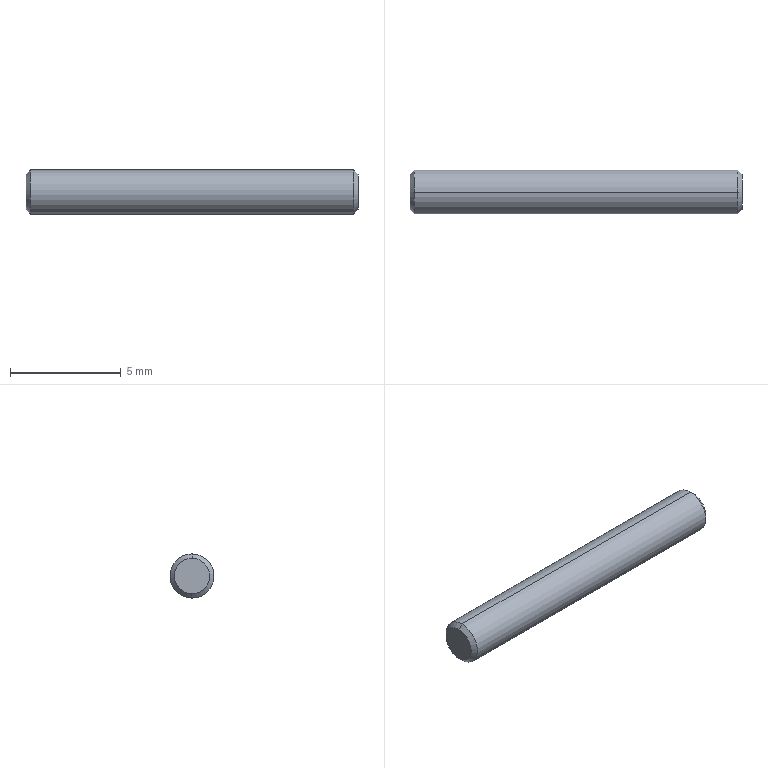Component | SolidWorks | F01AE00111-A2000-21TopEdgeAssembly-1_F01AE00111-A2000-19TopEdgeRollerAssembly-1_PIN 2X15--1 | 1 solid | 8 faces | box 15 x 2 x 2 mm | volume 47 mm3 | cone 4 | cylinder 2 | plane 2 | commonest cylinder face diameters 2 x2
build123d program:
from build123d import *

# Parameters (mm, degrees)
SKETCH1_R           = 1
BOSS_EXTRUDE1_DEPTH = 15
CHAMFER1_SIZE       = 0.2


with BuildPart() as part:
    # Sketch1 → Boss-Extrude1 (new body)
    with BuildSketch(Plane(origin=(0, 0, 0), x_dir=(1, 0, 0), z_dir=(0, 1, 0))):
        with Locations(Location((0, 0, 0), (0, 0, 270))):
            Circle(SKETCH1_R)
    extrude(amount=BOSS_EXTRUDE1_DEPTH)

    # Chamfer1
    chamfer1_edges = [part.edges().sort_by_distance(p)[0] for p in [
        (0, 0, -1),
        (0, 15, -1),
    ]]
    chamfer(chamfer1_edges, length=CHAMFER1_SIZE)


solid = part.part

# Placed as in the assembly
solid = solid.moved(Location((-133.352, 83.898, -383.475), (0, 0, 90)))
STEP:
#1=CARTESIAN_POINT('',(-5.841,3.303,-15.129));
#2=VERTEX_POINT('',#1);
#3=CARTESIAN_POINT('',(-5.841,3.303,-15.066));
#4=VERTEX_POINT('',#3);
#5=CARTESIAN_POINT('',(-5.841,3.303,-15.097));
#6=DIRECTION('',(-1.,-0.,-0.));
#7=DIRECTION('',(0.,0.01052,-0.9999));
#8=AXIS2_PLACEMENT_3D('',#5,#6,#7);
#9=CIRCLE('',#8,0.0315);
#10=EDGE_CURVE('',#2,#4,#9,.T.);
#11=ORIENTED_EDGE('',*,*,#10,.F.);
#12=CARTESIAN_POINT('',(-5.833,3.303,-15.137));
#13=VERTEX_POINT('',#12);
#14=CARTESIAN_POINT('',(-5.841,3.303,-15.129));
#15=DIRECTION('',(0.7071,0.00744,-0.7071));
#16=VECTOR('',#15,39.37);
#17=LINE('',#14,#16);
#18=EDGE_CURVE('',#2,#13,#17,.T.);
#19=ORIENTED_EDGE('',*,*,#18,.T.);
#20=CARTESIAN_POINT('',(-5.833,3.303,-15.058));
#21=VERTEX_POINT('',#20);
#22=CARTESIAN_POINT('',(-5.833,3.303,-15.097));
#23=DIRECTION('',(1.,0.,0.));
#24=DIRECTION('',(0.,0.01052,-0.9999));
#25=AXIS2_PLACEMENT_3D('',#22,#23,#24);
#26=CIRCLE('',#25,0.03937);
#27=EDGE_CURVE('',#21,#13,#26,.T.);
#28=ORIENTED_EDGE('',*,*,#27,.F.);
#29=CARTESIAN_POINT('',(-5.841,3.303,-15.066));
#30=DIRECTION('',(0.7071,-0.00744,0.7071));
#31=VECTOR('',#30,39.37);
#32=LINE('',#29,#31);
#33=EDGE_CURVE('',#4,#21,#32,.T.);
#34=ORIENTED_EDGE('',*,*,#33,.F.);
#35=EDGE_LOOP('',(#11,#19,#28,#34));
#36=FACE_OUTER_BOUND('',#35,.T.);
#37=CARTESIAN_POINT('',(-5.841,3.303,-15.097));
#38=DIRECTION('',(1.,0.,0.));
#39=DIRECTION('',(0.,-0.01052,0.9999));
#40=AXIS2_PLACEMENT_3D('',#37,#38,#39);
#41=CONICAL_SURFACE('',#40,0.0315,0.7854);
#42=ADVANCED_FACE('',(#36),#41,.T.);
#43=CARTESIAN_POINT('',(-5.25,3.303,-15.066));
#44=VERTEX_POINT('',#43);
#45=CARTESIAN_POINT('',(-5.25,3.303,-15.129));
#46=VERTEX_POINT('',#45);
#47=CARTESIAN_POINT('',(-5.25,3.303,-15.097));
#48=DIRECTION('',(1.,0.,0.));
#49=DIRECTION('',(0.,0.01052,-0.9999));
#50=AXIS2_PLACEMENT_3D('',#47,#48,#49);
#51=CIRCLE('',#50,0.0315);
#52=EDGE_CURVE('',#44,#46,#51,.T.);
#53=ORIENTED_EDGE('',*,*,#52,.F.);
#54=CARTESIAN_POINT('',(-5.258,3.303,-15.058));
#55=VERTEX_POINT('',#54);
#56=CARTESIAN_POINT('',(-5.258,3.303,-15.058));
#57=DIRECTION('',(-0.7071,-0.00744,0.7071));
#58=VECTOR('',#57,39.37);
#59=LINE('',#56,#58);
#60=EDGE_CURVE('',#44,#55,#59,.T.);
#61=ORIENTED_EDGE('',*,*,#60,.T.);
#62=CARTESIAN_POINT('',(-5.258,3.303,-15.137));
#63=VERTEX_POINT('',#62);
#64=CARTESIAN_POINT('',(-5.258,3.303,-15.097));
#65=DIRECTION('',(-1.,-0.,-0.));
#66=DIRECTION('',(0.,0.01052,-0.9999));
#67=AXIS2_PLACEMENT_3D('',#64,#65,#66);
#68=CIRCLE('',#67,0.03937);
#69=EDGE_CURVE('',#63,#55,#68,.T.);
#70=ORIENTED_EDGE('',*,*,#69,.F.);
#71=CARTESIAN_POINT('',(-5.258,3.303,-15.137));
#72=DIRECTION('',(-0.7071,0.00744,-0.7071));
#73=VECTOR('',#72,39.37);
#74=LINE('',#71,#73);
#75=EDGE_CURVE('',#46,#63,#74,.T.);
#76=ORIENTED_EDGE('',*,*,#75,.F.);
#77=EDGE_LOOP('',(#53,#61,#70,#76));
#78=FACE_OUTER_BOUND('',#77,.T.);
#79=CARTESIAN_POINT('',(-5.258,3.303,-15.097));
#80=DIRECTION('',(-1.,-0.,-0.));
#81=DIRECTION('',(0.,0.01052,-0.9999));
#82=AXIS2_PLACEMENT_3D('',#79,#80,#81);
#83=CONICAL_SURFACE('',#82,0.03937,0.7854);
#84=ADVANCED_FACE('',(#78),#83,.T.);
#85=ORIENTED_EDGE('',*,*,#27,.T.);
#86=CARTESIAN_POINT('',(-5.841,3.303,-15.137));
#87=DIRECTION('',(1.,0.,0.));
#88=VECTOR('',#87,39.37);
#89=LINE('',#86,#88);
#90=EDGE_CURVE('',#13,#63,#89,.T.);
#91=ORIENTED_EDGE('',*,*,#90,.T.);
#92=ORIENTED_EDGE('',*,*,#69,.T.);
#93=CARTESIAN_POINT('',(-5.841,3.303,-15.058));
#94=DIRECTION('',(1.,0.,0.));
#95=VECTOR('',#94,39.37);
#96=LINE('',#93,#95);
#97=EDGE_CURVE('',#21,#55,#96,.T.);
#98=ORIENTED_EDGE('',*,*,#97,.F.);
#99=EDGE_LOOP('',(#85,#91,#92,#98));
#100=FACE_OUTER_BOUND('',#99,.T.);
#101=CARTESIAN_POINT('',(-5.841,3.303,-15.097));
#102=DIRECTION('',(1.,0.,0.));
#103=DIRECTION('',(0.,-0.01052,0.9999));
#104=AXIS2_PLACEMENT_3D('',#101,#102,#103);
#105=CYLINDRICAL_SURFACE('',#104,0.03937);
#106=ADVANCED_FACE('',(#100),#105,.T.);
#107=ORIENTED_EDGE('',*,*,#90,.F.);
#108=CARTESIAN_POINT('',(-5.833,3.303,-15.097));
#109=DIRECTION('',(1.,0.,0.));
#110=DIRECTION('',(0.,0.01052,-0.9999));
#111=AXIS2_PLACEMENT_3D('',#108,#109,#110);
#112=CIRCLE('',#111,0.03937);
#113=EDGE_CURVE('',#13,#21,#112,.T.);
#114=ORIENTED_EDGE('',*,*,#113,.T.);
#115=ORIENTED_EDGE('',*,*,#97,.T.);
#116=CARTESIAN_POINT('',(-5.258,3.303,-15.097));
#117=DIRECTION('',(-1.,-0.,-0.));
#118=DIRECTION('',(0.,0.01052,-0.9999));
#119=AXIS2_PLACEMENT_3D('',#116,#117,#118);
#120=CIRCLE('',#119,0.03937);
#121=EDGE_CURVE('',#55,#63,#120,.T.);
#122=ORIENTED_EDGE('',*,*,#121,.T.);
#123=EDGE_LOOP('',(#107,#114,#115,#122));
#124=FACE_OUTER_BOUND('',#123,.T.);
#125=CARTESIAN_POINT('',(-5.841,3.303,-15.097));
#126=DIRECTION('',(1.,0.,0.));
#127=DIRECTION('',(0.,-0.01052,0.9999));
#128=AXIS2_PLACEMENT_3D('',#125,#126,#127);
#129=CYLINDRICAL_SURFACE('',#128,0.03937);
#130=ADVANCED_FACE('',(#124),#129,.T.);
#131=CARTESIAN_POINT('',(-5.841,3.303,-15.097));
#132=DIRECTION('',(-1.,-0.,-0.));
#133=DIRECTION('',(0.,0.01052,-0.9999));
#134=AXIS2_PLACEMENT_3D('',#131,#132,#133);
#135=CIRCLE('',#134,0.0315);
#136=EDGE_CURVE('',#4,#2,#135,.T.);
#137=ORIENTED_EDGE('',*,*,#136,.T.);
#138=ORIENTED_EDGE('',*,*,#10,.T.);
#139=EDGE_LOOP('',(#137,#138));
#140=FACE_OUTER_BOUND('',#139,.T.);
#141=CARTESIAN_POINT('',(-5.841,3.303,-15.097));
#142=DIRECTION('',(-1.,-0.,-0.));
#143=DIRECTION('',(0.,0.01052,-0.9999));
#144=AXIS2_PLACEMENT_3D('',#141,#142,#143);
#145=PLANE('',#144);
#146=ADVANCED_FACE('',(#140),#145,.T.);
#147=CARTESIAN_POINT('',(-5.25,3.303,-15.097));
#148=DIRECTION('',(1.,0.,0.));
#149=DIRECTION('',(0.,0.01052,-0.9999));
#150=AXIS2_PLACEMENT_3D('',#147,#148,#149);
#151=CIRCLE('',#150,0.0315);
#152=EDGE_CURVE('',#46,#44,#151,.T.);
#153=ORIENTED_EDGE('',*,*,#152,.T.);
#154=ORIENTED_EDGE('',*,*,#52,.T.);
#155=EDGE_LOOP('',(#153,#154));
#156=FACE_OUTER_BOUND('',#155,.T.);
#157=CARTESIAN_POINT('',(-5.25,3.303,-15.097));
#158=DIRECTION('',(-1.,-0.,-0.));
#159=DIRECTION('',(0.,0.01052,-0.9999));
#160=AXIS2_PLACEMENT_3D('',#157,#158,#159);
#161=PLANE('',#160);
#162=ADVANCED_FACE('',(#156),#161,.F.);
#163=ORIENTED_EDGE('',*,*,#60,.F.);
#164=ORIENTED_EDGE('',*,*,#152,.F.);
#165=ORIENTED_EDGE('',*,*,#75,.T.);
#166=ORIENTED_EDGE('',*,*,#121,.F.);
#167=EDGE_LOOP('',(#163,#164,#165,#166));
#168=FACE_OUTER_BOUND('',#167,.T.);
#169=CARTESIAN_POINT('',(-5.258,3.303,-15.097));
#170=DIRECTION('',(-1.,-0.,-0.));
#171=DIRECTION('',(0.,0.01052,-0.9999));
#172=AXIS2_PLACEMENT_3D('',#169,#170,#171);
#173=CONICAL_SURFACE('',#172,0.03937,0.7854);
#174=ADVANCED_FACE('',(#168),#173,.T.);
#175=ORIENTED_EDGE('',*,*,#18,.F.);
#176=ORIENTED_EDGE('',*,*,#136,.F.);
#177=ORIENTED_EDGE('',*,*,#33,.T.);
#178=ORIENTED_EDGE('',*,*,#113,.F.);
#179=EDGE_LOOP('',(#175,#176,#177,#178));
#180=FACE_OUTER_BOUND('',#179,.T.);
#181=CARTESIAN_POINT('',(-5.841,3.303,-15.097));
#182=DIRECTION('',(1.,0.,0.));
#183=DIRECTION('',(0.,-0.01052,0.9999));
#184=AXIS2_PLACEMENT_3D('',#181,#182,#183);
#185=CONICAL_SURFACE('',#184,0.0315,0.7854);
#186=ADVANCED_FACE('',(#180),#185,.T.);
#187=CLOSED_SHELL('',(#42,#84,#106,#130,#146,#162,#174,#186));
#188=MANIFOLD_SOLID_BREP('',#187);
#189=CARTESIAN_POINT('',(0.,0.,0.));
#190=DIRECTION('',(0.,0.,1.));
#191=DIRECTION('',(1.,0.,0.));
#192=AXIS2_PLACEMENT_3D('',#189,#190,#191);
#193=(LENGTH_UNIT()NAMED_UNIT(*)SI_UNIT($,.METRE.));
#194=LENGTH_MEASURE_WITH_UNIT(LENGTH_MEASURE(0.0254),#193);
#195=DIMENSIONAL_EXPONENTS(1.,0.,0.,0.,0.,0.,0.);
#196=(CONVERSION_BASED_UNIT('',#194)LENGTH_UNIT()NAMED_UNIT(#195));
#197=UNCERTAINTY_MEASURE_WITH_UNIT(LENGTH_MEASURE(0.00001),#196,'','');
#198=(NAMED_UNIT(*)PLANE_ANGLE_UNIT()SI_UNIT($,.RADIAN.));
#199=(NAMED_UNIT(*)SI_UNIT($,.STERADIAN.)SOLID_ANGLE_UNIT());
#200=(GEOMETRIC_REPRESENTATION_CONTEXT(3)GLOBAL_UNCERTAINTY_ASSIGNED_CONTEXT((#197))GLOBAL_UNIT_ASSIGNED_CONTEXT((#196,#198,#199))REPRESENTATION_CONTEXT('',''));
#201=ADVANCED_BREP_SHAPE_REPRESENTATION('',(#188,#192),#200);
#202=COLOUR_RGB('',0.7922,0.8196,0.9333);
#203=FILL_AREA_STYLE_COLOUR('',#202);
#204=FILL_AREA_STYLE('',(#203));
#205=SURFACE_STYLE_FILL_AREA(#204);
#206=SURFACE_SIDE_STYLE('',(#205));
#207=SURFACE_STYLE_USAGE(.BOTH.,#206);
#208=PRESENTATION_STYLE_ASSIGNMENT((#207));
#209=STYLED_ITEM('',(#208),#188);
#210=(LENGTH_UNIT()NAMED_UNIT(*)SI_UNIT($,.METRE.));
#211=LENGTH_MEASURE_WITH_UNIT(LENGTH_MEASURE(0.0254),#210);
#212=DIMENSIONAL_EXPONENTS(1.,0.,0.,0.,0.,0.,0.);
#213=(CONVERSION_BASED_UNIT('',#211)LENGTH_UNIT()NAMED_UNIT(#212));
#214=UNCERTAINTY_MEASURE_WITH_UNIT(LENGTH_MEASURE(0.00001),#213,'','');
#215=(NAMED_UNIT(*)PLANE_ANGLE_UNIT()SI_UNIT($,.RADIAN.));
#216=(NAMED_UNIT(*)SI_UNIT($,.STERADIAN.)SOLID_ANGLE_UNIT());
#217=(GEOMETRIC_REPRESENTATION_CONTEXT(3)GLOBAL_UNCERTAINTY_ASSIGNED_CONTEXT((#214))GLOBAL_UNIT_ASSIGNED_CONTEXT((#213,#215,#216))REPRESENTATION_CONTEXT('',''));
#218=MECHANICAL_DESIGN_GEOMETRIC_PRESENTATION_REPRESENTATION('',(#209),#217);
#219=PRESENTATION_LAYER_ASSIGNMENT('','',(#209));